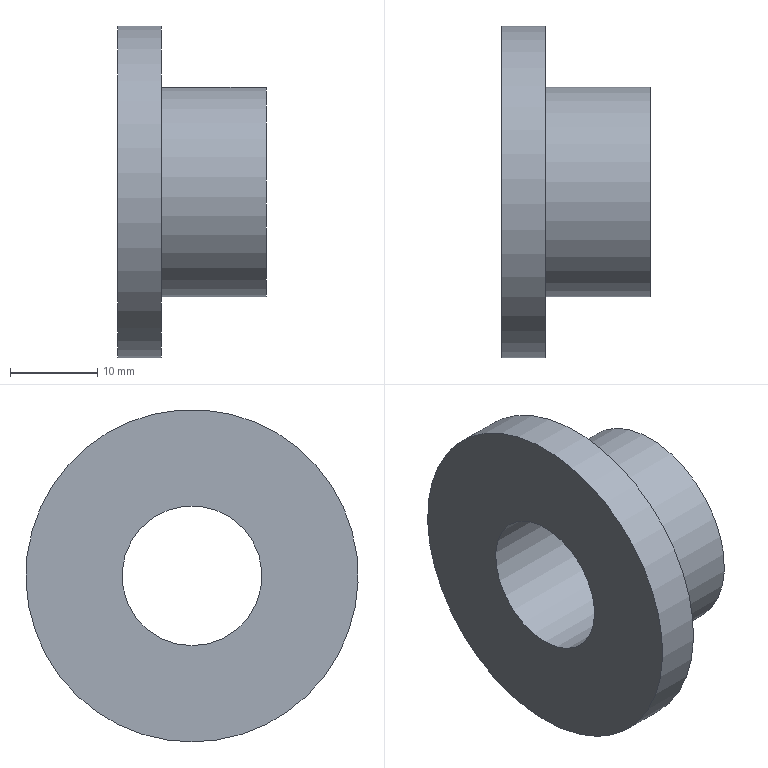Component | NX | PACKING_GLAND | 1 solid | 6 faces | box 17 x 38 x 38 mm | volume 7212 mm3 | cylinder 3 | plane 2 | cone 1 | commonest cylinder face diameters 16 x1 24 x1 38 x1
STEP:
#1=CARTESIAN_POINT('',(0.,0.,0.));
#2=DIRECTION('',(0.,0.,1.));
#3=DIRECTION('',(1.,0.,0.));
#4=AXIS2_PLACEMENT_3D('',#1,#2,#3);
#5=CARTESIAN_POINT('',(-9.288,0.,-8.));
#6=VERTEX_POINT('',#5);
#7=CARTESIAN_POINT('',(-9.288,0.,0.));
#8=DIRECTION('',(-1.,0.,0.));
#9=DIRECTION('',(0.,0.,-1.));
#10=AXIS2_PLACEMENT_3D('',#7,#8,#9);
#11=CIRCLE('',#10,8.);
#12=CARTESIAN_POINT('',(-9.288,0.,19.));
#13=DIRECTION('',(1.,0.,0.));
#14=DIRECTION('',(0.,0.,1.));
#15=AXIS2_PLACEMENT_3D('',#12,#13,#14);
#16=PLANE('',#15);
#17=CARTESIAN_POINT('',(-27.,0.));
#18=CARTESIAN_POINT('',(-27.,13.856));
#19=CARTESIAN_POINT('',(-15.,6.928));
#20=CARTESIAN_POINT('',(-3.,0.));
#21=CARTESIAN_POINT('',(-15.,-6.928));
#22=CARTESIAN_POINT('',(-27.,-13.856));
#23=CARTESIAN_POINT('',(-27.,0.));
#24=(BOUNDED_CURVE()B_SPLINE_CURVE(2,(#17,#18,#19,#20,#21,#22,#23),.UNSPECIFIED.,.T.,.F.)B_SPLINE_CURVE_WITH_KNOTS((1,2,2,2,2,1),(-2.094,0.,2.094,4.189,6.283,8.378),.UNSPECIFIED.)CURVE()GEOMETRIC_REPRESENTATION_ITEM()RATIONAL_B_SPLINE_CURVE((1.,0.5,1.,0.5,1.,0.5,1.))REPRESENTATION_ITEM(''));
#25=(GEOMETRIC_REPRESENTATION_CONTEXT(2)PARAMETRIC_REPRESENTATION_CONTEXT()REPRESENTATION_CONTEXT('',''));
#26=DEFINITIONAL_REPRESENTATION('',(#24),#25);
#27=PCURVE('',#16,#26);
#28=CARTESIAN_POINT('',(7.712,0.,0.));
#29=DIRECTION('',(-1.,0.,0.));
#30=DIRECTION('',(0.,0.,-1.));
#31=AXIS2_PLACEMENT_3D('',#28,#29,#30);
#32=CYLINDRICAL_SURFACE('',#31,8.);
#33=CARTESIAN_POINT('',(0.,17.));
#34=DIRECTION('',(1.,0.));
#35=VECTOR('',#34,1.);
#36=LINE('',#33,#35);
#37=(GEOMETRIC_REPRESENTATION_CONTEXT(2)PARAMETRIC_REPRESENTATION_CONTEXT()REPRESENTATION_CONTEXT('',''));
#38=DEFINITIONAL_REPRESENTATION('',(#36),#37);
#39=PCURVE('',#32,#38);
#40=SURFACE_CURVE('',#11,(#27,#39),.PCURVE_S1.);
#41=EDGE_CURVE('',#6,#6,#40,.T.);
#42=ORIENTED_EDGE('',*,*,#41,.F.);
#43=EDGE_LOOP('',(#42));
#44=FACE_BOUND('',#43,.T.);
#45=CARTESIAN_POINT('',(-9.288,0.,-19.));
#46=VERTEX_POINT('',#45);
#47=CARTESIAN_POINT('',(-9.288,0.,0.));
#48=DIRECTION('',(-1.,0.,0.));
#49=DIRECTION('',(0.,0.,-1.));
#50=AXIS2_PLACEMENT_3D('',#47,#48,#49);
#51=CIRCLE('',#50,19.);
#52=CARTESIAN_POINT('',(-38.,0.));
#53=CARTESIAN_POINT('',(-38.,32.909));
#54=CARTESIAN_POINT('',(-9.5,16.454));
#55=CARTESIAN_POINT('',(19.,0.));
#56=CARTESIAN_POINT('',(-9.5,-16.454));
#57=CARTESIAN_POINT('',(-38.,-32.909));
#58=CARTESIAN_POINT('',(-38.,0.));
#59=(BOUNDED_CURVE()B_SPLINE_CURVE(2,(#52,#53,#54,#55,#56,#57,#58),.UNSPECIFIED.,.T.,.F.)B_SPLINE_CURVE_WITH_KNOTS((1,2,2,2,2,1),(-2.094,0.,2.094,4.189,6.283,8.378),.UNSPECIFIED.)CURVE()GEOMETRIC_REPRESENTATION_ITEM()RATIONAL_B_SPLINE_CURVE((1.,0.5,1.,0.5,1.,0.5,1.))REPRESENTATION_ITEM(''));
#60=(GEOMETRIC_REPRESENTATION_CONTEXT(2)PARAMETRIC_REPRESENTATION_CONTEXT()REPRESENTATION_CONTEXT('',''));
#61=DEFINITIONAL_REPRESENTATION('',(#59),#60);
#62=PCURVE('',#16,#61);
#63=CARTESIAN_POINT('',(7.712,0.,0.));
#64=DIRECTION('',(-1.,0.,0.));
#65=DIRECTION('',(0.,0.,-1.));
#66=AXIS2_PLACEMENT_3D('',#63,#64,#65);
#67=CYLINDRICAL_SURFACE('',#66,19.);
#68=CARTESIAN_POINT('',(0.,17.));
#69=DIRECTION('',(1.,0.));
#70=VECTOR('',#69,1.);
#71=LINE('',#68,#70);
#72=(GEOMETRIC_REPRESENTATION_CONTEXT(2)PARAMETRIC_REPRESENTATION_CONTEXT()REPRESENTATION_CONTEXT('',''));
#73=DEFINITIONAL_REPRESENTATION('',(#71),#72);
#74=PCURVE('',#67,#73);
#75=SURFACE_CURVE('',#51,(#62,#74),.PCURVE_S1.);
#76=EDGE_CURVE('',#46,#46,#75,.T.);
#77=ORIENTED_EDGE('',*,*,#76,.T.);
#78=EDGE_LOOP('',(#77));
#79=FACE_BOUND('',#78,.T.);
#80=ADVANCED_FACE('',(#44,#79),#16,.F.);
#81=CARTESIAN_POINT('',(3.712,0.,-8.));
#82=VERTEX_POINT('',#81);
#83=CARTESIAN_POINT('',(3.712,0.,0.));
#84=DIRECTION('',(1.,0.,0.));
#85=DIRECTION('',(0.,0.,-1.));
#86=AXIS2_PLACEMENT_3D('',#83,#84,#85);
#87=CIRCLE('',#86,8.);
#88=CARTESIAN_POINT('',(6.283,4.));
#89=DIRECTION('',(-1.,0.));
#90=VECTOR('',#89,1.);
#91=LINE('',#88,#90);
#92=(GEOMETRIC_REPRESENTATION_CONTEXT(2)PARAMETRIC_REPRESENTATION_CONTEXT()REPRESENTATION_CONTEXT('',''));
#93=DEFINITIONAL_REPRESENTATION('',(#91),#92);
#94=PCURVE('',#32,#93);
#95=CARTESIAN_POINT('',(7.712,0.,0.));
#96=DIRECTION('',(1.,0.,0.));
#97=DIRECTION('',(0.,0.,1.));
#98=AXIS2_PLACEMENT_3D('',#95,#96,#97);
#99=CONICAL_SURFACE('',#98,12.,0.7854);
#100=CARTESIAN_POINT('',(3.142,-4.));
#101=DIRECTION('',(1.,0.));
#102=VECTOR('',#101,1.);
#103=LINE('',#100,#102);
#104=(GEOMETRIC_REPRESENTATION_CONTEXT(2)PARAMETRIC_REPRESENTATION_CONTEXT()REPRESENTATION_CONTEXT('',''));
#105=DEFINITIONAL_REPRESENTATION('',(#103),#104);
#106=PCURVE('',#99,#105);
#107=SURFACE_CURVE('',#87,(#94,#106),.PCURVE_S1.);
#108=EDGE_CURVE('',#82,#82,#107,.T.);
#109=ORIENTED_EDGE('',*,*,#108,.F.);
#110=CARTESIAN_POINT('',(3.712,0.,-8.));
#111=CARTESIAN_POINT('',(-9.288,0.,-8.));
#112=B_SPLINE_CURVE_WITH_KNOTS('',1,(#110,#111),.UNSPECIFIED.,.F.,.F.,(2,2),(4.,17.),.PIECEWISE_BEZIER_KNOTS.);
#113=CARTESIAN_POINT('',(6.283,0.));
#114=DIRECTION('',(0.,1.));
#115=VECTOR('',#114,1.);
#116=LINE('',#113,#115);
#117=(GEOMETRIC_REPRESENTATION_CONTEXT(2)PARAMETRIC_REPRESENTATION_CONTEXT()REPRESENTATION_CONTEXT('',''));
#118=DEFINITIONAL_REPRESENTATION('',(#116),#117);
#119=PCURVE('',#32,#118);
#120=CARTESIAN_POINT('',(0.,0.));
#121=DIRECTION('',(0.,1.));
#122=VECTOR('',#121,1.);
#123=LINE('',#120,#122);
#124=(GEOMETRIC_REPRESENTATION_CONTEXT(2)PARAMETRIC_REPRESENTATION_CONTEXT()REPRESENTATION_CONTEXT('',''));
#125=DEFINITIONAL_REPRESENTATION('',(#123),#124);
#126=PCURVE('',#32,#125);
#127=SEAM_CURVE('',#112,(#119,#126),.PCURVE_S1.);
#128=EDGE_CURVE('',#82,#6,#127,.T.);
#129=ORIENTED_EDGE('',*,*,#128,.T.);
#130=ORIENTED_EDGE('',*,*,#41,.F.);
#131=ORIENTED_EDGE('',*,*,#128,.F.);
#132=EDGE_LOOP('',(#109,#129,#130,#131));
#133=FACE_BOUND('',#132,.F.);
#134=ADVANCED_FACE('',(#133),#32,.F.);
#135=CARTESIAN_POINT('',(-4.288,0.,-12.));
#136=VERTEX_POINT('',#135);
#137=CARTESIAN_POINT('',(-4.288,0.,0.));
#138=DIRECTION('',(-1.,0.,0.));
#139=DIRECTION('',(0.,0.,-1.));
#140=AXIS2_PLACEMENT_3D('',#137,#138,#139);
#141=CIRCLE('',#140,12.);
#142=CARTESIAN_POINT('',(7.712,0.,0.));
#143=DIRECTION('',(-1.,0.,0.));
#144=DIRECTION('',(0.,0.,-1.));
#145=AXIS2_PLACEMENT_3D('',#142,#143,#144);
#146=CYLINDRICAL_SURFACE('',#145,12.);
#147=CARTESIAN_POINT('',(0.,12.));
#148=DIRECTION('',(1.,0.));
#149=VECTOR('',#148,1.);
#150=LINE('',#147,#149);
#151=(GEOMETRIC_REPRESENTATION_CONTEXT(2)PARAMETRIC_REPRESENTATION_CONTEXT()REPRESENTATION_CONTEXT('',''));
#152=DEFINITIONAL_REPRESENTATION('',(#150),#151);
#153=PCURVE('',#146,#152);
#154=CARTESIAN_POINT('',(-4.288,0.,12.));
#155=DIRECTION('',(-1.,0.,0.));
#156=DIRECTION('',(0.,0.,-1.));
#157=AXIS2_PLACEMENT_3D('',#154,#155,#156);
#158=PLANE('',#157);
#159=CARTESIAN_POINT('',(12.,0.));
#160=DIRECTION('',(1.,0.));
#161=AXIS2_PLACEMENT_2D('',#159,#160);
#162=CIRCLE('',#161,12.);
#163=(GEOMETRIC_REPRESENTATION_CONTEXT(2)PARAMETRIC_REPRESENTATION_CONTEXT()REPRESENTATION_CONTEXT('',''));
#164=DEFINITIONAL_REPRESENTATION('',(#162),#163);
#165=PCURVE('',#158,#164);
#166=SURFACE_CURVE('',#141,(#153,#165),.PCURVE_S1.);
#167=EDGE_CURVE('',#136,#136,#166,.T.);
#168=ORIENTED_EDGE('',*,*,#167,.F.);
#169=CARTESIAN_POINT('',(7.712,0.,-12.));
#170=VERTEX_POINT('',#169);
#171=CARTESIAN_POINT('',(7.712,0.,-12.));
#172=CARTESIAN_POINT('',(-4.288,0.,-12.));
#173=B_SPLINE_CURVE_WITH_KNOTS('',1,(#171,#172),.UNSPECIFIED.,.F.,.F.,(2,2),(0.,12.),.PIECEWISE_BEZIER_KNOTS.);
#174=CARTESIAN_POINT('',(0.,0.));
#175=DIRECTION('',(0.,1.));
#176=VECTOR('',#175,1.);
#177=LINE('',#174,#176);
#178=(GEOMETRIC_REPRESENTATION_CONTEXT(2)PARAMETRIC_REPRESENTATION_CONTEXT()REPRESENTATION_CONTEXT('',''));
#179=DEFINITIONAL_REPRESENTATION('',(#177),#178);
#180=PCURVE('',#146,#179);
#181=CARTESIAN_POINT('',(6.283,0.));
#182=DIRECTION('',(0.,1.));
#183=VECTOR('',#182,1.);
#184=LINE('',#181,#183);
#185=(GEOMETRIC_REPRESENTATION_CONTEXT(2)PARAMETRIC_REPRESENTATION_CONTEXT()REPRESENTATION_CONTEXT('',''));
#186=DEFINITIONAL_REPRESENTATION('',(#184),#185);
#187=PCURVE('',#146,#186);
#188=SEAM_CURVE('',#173,(#180,#187),.PCURVE_S1.);
#189=EDGE_CURVE('',#170,#136,#188,.T.);
#190=ORIENTED_EDGE('',*,*,#189,.F.);
#191=CARTESIAN_POINT('',(7.712,0.,0.));
#192=DIRECTION('',(-1.,0.,0.));
#193=DIRECTION('',(0.,0.,-1.));
#194=AXIS2_PLACEMENT_3D('',#191,#192,#193);
#195=CIRCLE('',#194,12.);
#196=CARTESIAN_POINT('',(0.,0.));
#197=DIRECTION('',(1.,0.));
#198=VECTOR('',#197,1.);
#199=LINE('',#196,#198);
#200=(GEOMETRIC_REPRESENTATION_CONTEXT(2)PARAMETRIC_REPRESENTATION_CONTEXT()REPRESENTATION_CONTEXT('',''));
#201=DEFINITIONAL_REPRESENTATION('',(#199),#200);
#202=PCURVE('',#146,#201);
#203=CARTESIAN_POINT('',(9.425,0.));
#204=DIRECTION('',(-1.,0.));
#205=VECTOR('',#204,1.);
#206=LINE('',#203,#205);
#207=(GEOMETRIC_REPRESENTATION_CONTEXT(2)PARAMETRIC_REPRESENTATION_CONTEXT()REPRESENTATION_CONTEXT('',''));
#208=DEFINITIONAL_REPRESENTATION('',(#206),#207);
#209=PCURVE('',#99,#208);
#210=SURFACE_CURVE('',#195,(#202,#209),.PCURVE_S1.);
#211=EDGE_CURVE('',#170,#170,#210,.T.);
#212=ORIENTED_EDGE('',*,*,#211,.T.);
#213=ORIENTED_EDGE('',*,*,#189,.T.);
#214=EDGE_LOOP('',(#168,#190,#212,#213));
#215=FACE_BOUND('',#214,.T.);
#216=ADVANCED_FACE('',(#215),#146,.T.);
#217=CARTESIAN_POINT('',(-4.288,0.,-19.));
#218=VERTEX_POINT('',#217);
#219=CARTESIAN_POINT('',(-4.288,0.,0.));
#220=DIRECTION('',(-1.,0.,0.));
#221=DIRECTION('',(0.,0.,-1.));
#222=AXIS2_PLACEMENT_3D('',#219,#220,#221);
#223=CIRCLE('',#222,19.);
#224=CARTESIAN_POINT('',(12.,0.));
#225=DIRECTION('',(1.,0.));
#226=AXIS2_PLACEMENT_2D('',#224,#225);
#227=CIRCLE('',#226,19.);
#228=(GEOMETRIC_REPRESENTATION_CONTEXT(2)PARAMETRIC_REPRESENTATION_CONTEXT()REPRESENTATION_CONTEXT('',''));
#229=DEFINITIONAL_REPRESENTATION('',(#227),#228);
#230=PCURVE('',#158,#229);
#231=CARTESIAN_POINT('',(0.,12.));
#232=DIRECTION('',(1.,0.));
#233=VECTOR('',#232,1.);
#234=LINE('',#231,#233);
#235=(GEOMETRIC_REPRESENTATION_CONTEXT(2)PARAMETRIC_REPRESENTATION_CONTEXT()REPRESENTATION_CONTEXT('',''));
#236=DEFINITIONAL_REPRESENTATION('',(#234),#235);
#237=PCURVE('',#67,#236);
#238=SURFACE_CURVE('',#223,(#230,#237),.PCURVE_S1.);
#239=EDGE_CURVE('',#218,#218,#238,.T.);
#240=ORIENTED_EDGE('',*,*,#239,.F.);
#241=EDGE_LOOP('',(#240));
#242=FACE_BOUND('',#241,.T.);
#243=ORIENTED_EDGE('',*,*,#167,.T.);
#244=EDGE_LOOP('',(#243));
#245=FACE_BOUND('',#244,.T.);
#246=ADVANCED_FACE('',(#242,#245),#158,.F.);
#247=ORIENTED_EDGE('',*,*,#76,.F.);
#248=CARTESIAN_POINT('',(-4.288,0.,-19.));
#249=CARTESIAN_POINT('',(-9.288,0.,-19.));
#250=B_SPLINE_CURVE_WITH_KNOTS('',1,(#248,#249),.UNSPECIFIED.,.F.,.F.,(2,2),(12.,17.),.PIECEWISE_BEZIER_KNOTS.);
#251=CARTESIAN_POINT('',(0.,0.));
#252=DIRECTION('',(0.,1.));
#253=VECTOR('',#252,1.);
#254=LINE('',#251,#253);
#255=(GEOMETRIC_REPRESENTATION_CONTEXT(2)PARAMETRIC_REPRESENTATION_CONTEXT()REPRESENTATION_CONTEXT('',''));
#256=DEFINITIONAL_REPRESENTATION('',(#254),#255);
#257=PCURVE('',#67,#256);
#258=CARTESIAN_POINT('',(6.283,0.));
#259=DIRECTION('',(0.,1.));
#260=VECTOR('',#259,1.);
#261=LINE('',#258,#260);
#262=(GEOMETRIC_REPRESENTATION_CONTEXT(2)PARAMETRIC_REPRESENTATION_CONTEXT()REPRESENTATION_CONTEXT('',''));
#263=DEFINITIONAL_REPRESENTATION('',(#261),#262);
#264=PCURVE('',#67,#263);
#265=SEAM_CURVE('',#250,(#257,#264),.PCURVE_S1.);
#266=EDGE_CURVE('',#218,#46,#265,.T.);
#267=ORIENTED_EDGE('',*,*,#266,.F.);
#268=ORIENTED_EDGE('',*,*,#239,.T.);
#269=ORIENTED_EDGE('',*,*,#266,.T.);
#270=EDGE_LOOP('',(#247,#267,#268,#269));
#271=FACE_BOUND('',#270,.T.);
#272=ADVANCED_FACE('',(#271),#67,.T.);
#273=ORIENTED_EDGE('',*,*,#108,.T.);
#274=CARTESIAN_POINT('',(3.712,-0.,-8.));
#275=CARTESIAN_POINT('',(7.712,-0.,-12.));
#276=B_SPLINE_CURVE_WITH_KNOTS('',1,(#274,#275),.UNSPECIFIED.,.F.,.F.,(2,2),(-5.657,0.),.PIECEWISE_BEZIER_KNOTS.);
#277=CARTESIAN_POINT('',(9.425,0.));
#278=DIRECTION('',(0.,1.));
#279=VECTOR('',#278,1.);
#280=LINE('',#277,#279);
#281=(GEOMETRIC_REPRESENTATION_CONTEXT(2)PARAMETRIC_REPRESENTATION_CONTEXT()REPRESENTATION_CONTEXT('',''));
#282=DEFINITIONAL_REPRESENTATION('',(#280),#281);
#283=PCURVE('',#99,#282);
#284=CARTESIAN_POINT('',(3.142,0.));
#285=DIRECTION('',(0.,1.));
#286=VECTOR('',#285,1.);
#287=LINE('',#284,#286);
#288=(GEOMETRIC_REPRESENTATION_CONTEXT(2)PARAMETRIC_REPRESENTATION_CONTEXT()REPRESENTATION_CONTEXT('',''));
#289=DEFINITIONAL_REPRESENTATION('',(#287),#288);
#290=PCURVE('',#99,#289);
#291=SEAM_CURVE('',#276,(#283,#290),.PCURVE_S1.);
#292=EDGE_CURVE('',#82,#170,#291,.T.);
#293=ORIENTED_EDGE('',*,*,#292,.T.);
#294=ORIENTED_EDGE('',*,*,#211,.T.);
#295=ORIENTED_EDGE('',*,*,#292,.F.);
#296=EDGE_LOOP('',(#273,#293,#294,#295));
#297=FACE_BOUND('',#296,.F.);
#298=ADVANCED_FACE('',(#297),#99,.F.);
#299=CLOSED_SHELL('',(#80,#134,#216,#246,#272,#298));
#300=MANIFOLD_SOLID_BREP('',#299);
#301=(LENGTH_UNIT()NAMED_UNIT(*)SI_UNIT(.MILLI.,.METRE.));
#302=UNCERTAINTY_MEASURE_WITH_UNIT(LENGTH_MEASURE(0.00001),#301,'','');
#303=(NAMED_UNIT(*)PLANE_ANGLE_UNIT()SI_UNIT($,.RADIAN.));
#304=(NAMED_UNIT(*)SI_UNIT($,.STERADIAN.)SOLID_ANGLE_UNIT());
#305=(GEOMETRIC_REPRESENTATION_CONTEXT(3)GLOBAL_UNCERTAINTY_ASSIGNED_CONTEXT((#302))GLOBAL_UNIT_ASSIGNED_CONTEXT((#301,#303,#304))REPRESENTATION_CONTEXT('',''));
#306=ADVANCED_BREP_SHAPE_REPRESENTATION('',(#4,#300),#305);